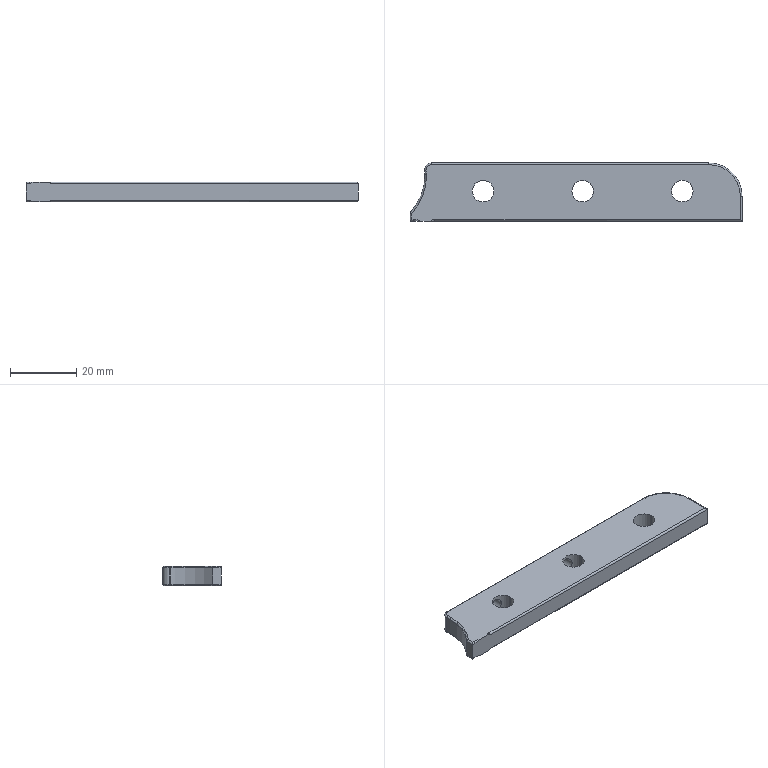Component | SolidWorks | Assembly5.1-1_TailstockAdjustmentPlate.1-1 | 1 solid | 42 faces | box 100 x 17.5 x 6 mm | volume 9302 mm3 | cylinder 24 | torus 12 | plane 6 | commonest cylinder face diameters 1 x10 4 x6 6.5 x6 20 x1 34 x1
build123d program:
from build123d import *

# Parameters (mm, degrees)
SKETCH1_2_R           = 3.25
BOSS_EXTRUDE1_DEPTH   = 6
M4_TAPPED_HOLE1_D     = 4
M4_TAPPED_HOLE1_DEPTH = 9
M4_TAPPED_HOLE1_TIP   = 1.202
FILLET1_R             = 0.5
SKETCH1_W             = 8.5
SKETCH1_H             = 3
CUT_EXTRUDE1_DEPTH    = 25


with BuildPart() as part:
    # Sketch1_2 → Boss-Extrude1 (new body)
    with BuildSketch(Plane.XY):
        with BuildLine():
            Line((-100, 0), (-100, 2.478))
            ThreePointArc((-100, 2.478), (-96.433, 8.446), (-95.553, 15.342))
            ThreePointArc((-95.553, 15.342), (-95.028, 16.857), (-93.559, 17.5))
            Line((-93.559, 17.5), (-10, 17.5))
            ThreePointArc((-10, 17.5), (-2.929, 14.571), (0, 7.5))
            Line((0, 7.5), (0, 0))
            Line((0, 0), (-92.5, 0))
            ThreePointArc((-92.5, 0), (-93.207, -0.2929), (-93.5, -1))
            Line((-93.5, -1), (-93.5, -2.5))
            Line((-93.5, -2.5), (-94.67, -2.5))
            ThreePointArc((-94.67, -2.5), (-96.5, -0.6699), (-99, 0))
            Line((-99, 0), (-100, 0))
        make_face()
        with Locations((-18, 9)):
            Circle(SKETCH1_2_R, mode=Mode.SUBTRACT)
        with Locations((-48, 9)):
            Circle(SKETCH1_2_R, mode=Mode.SUBTRACT)
        with Locations((-78, 9)):
            Circle(SKETCH1_2_R, mode=Mode.SUBTRACT)
    extrude(amount=BOSS_EXTRUDE1_DEPTH)

    # M4 Tapped Hole1
    with Locations(Plane(origin=(0, 17.5, 0), x_dir=(-1, 0, 0), z_dir=(0, 1, 0))):
        with Locations((48, 3), (78, 3)):
            Hole(M4_TAPPED_HOLE1_D / 2, depth=M4_TAPPED_HOLE1_DEPTH)
            with Locations((0, 0, -(M4_TAPPED_HOLE1_DEPTH + M4_TAPPED_HOLE1_TIP / 2))):  # 118° drill point
                Cone(0, M4_TAPPED_HOLE1_D / 2, M4_TAPPED_HOLE1_TIP, mode=Mode.SUBTRACT)

    # Fillet1
    fillet1_edges = [part.edges().sort_by_distance(p)[0] for p in [
        (-51.78, 17.5, 6),
        (-46.25, 0, 0),
        (-93.207, -0.2929, 0),
        (-93.5, -1.75, 0),
        (-94.085, -2.5, 0),
        (-96.5, -0.6699, 0),
        (-99.5, 0, 0),
        (-95.028, 16.857, 6),
        (-100, 1.239, 0),
        (-96.433, 8.446, 0),
        (-95.028, 16.857, 0),
        (-51.78, 17.5, 0),
        (-2.929, 14.571, 0),
        (0, 3.75, 0),
        (-96.433, 8.446, 6),
        (-100, 1.239, 6),
        (-99.5, 0, 6),
        (-96.5, -0.6699, 6),
        (-94.085, -2.5, 6),
        (-93.5, -1.75, 6),
        (-93.207, -0.2929, 6),
        (-46.25, 0, 6),
        (0, 3.75, 6),
        (-2.929, 14.571, 6),
    ]]
    fillet(fillet1_edges, radius=FILLET1_R)

    # Sketch1 → Cut-Extrude1 (cut, symmetric)
    with BuildSketch(Plane.XY):
        with Locations((-96.75, -1.5)):
            Rectangle(SKETCH1_W, SKETCH1_H)
    extrude(amount=CUT_EXTRUDE1_DEPTH, both=True, mode=Mode.SUBTRACT)


solid = part.part

# Placed as in the assembly
solid = solid.moved(Location((238, 136, 7.563), (0, 0, 0)))